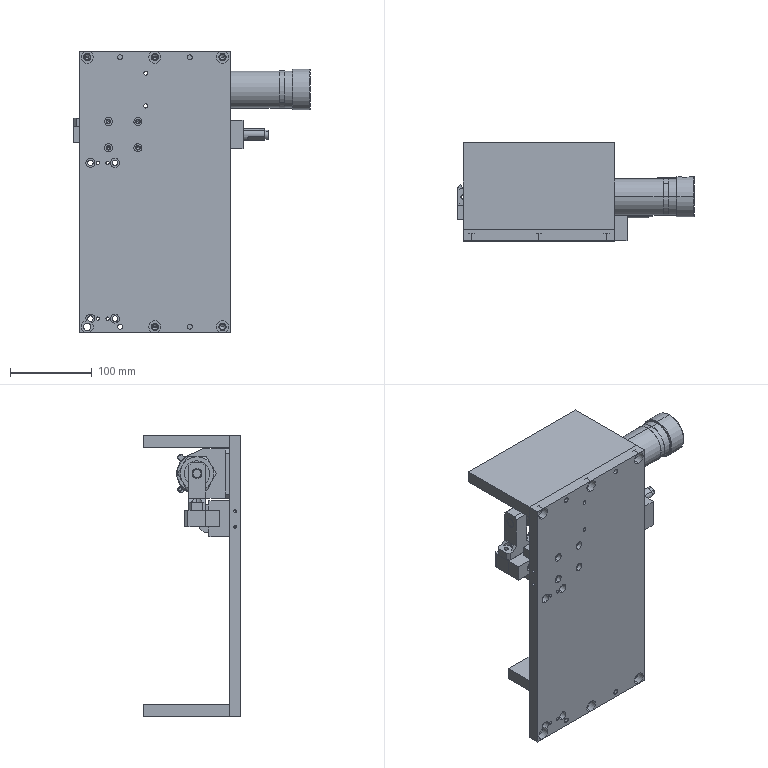Assembly | SolidWorks | mm | 19 component files | 19 solids | 807 faces | box 288.5 x 119.4 x 344 mm | volume 1839364 mm3 | plane 357 | cylinder 309 | cone 109 | torus 28 | sphere 4 | commonest cylinder face diameters 6.8 x26 6 x26 10 x18 5.5 x18 4.2 x18 11 x14 21.289 x14 45 x12
Bill of materials:
40_M12x1_25_Nut | 1 |  | Hexagonal prism with a central cylindrical through-bore and chamfered corners on both faces; looks like a hex nut.
ACA_1412_1_NT | 2 |  | Thin hexagonal prism with a large central through-bore and chamfered edges; looks like a thin hex nut or a hex ring.
ACA_1412_2_N_Body | 1 |  | Long stepped cylindrical body: a small-diameter pin at one end, narrow circumferential grooves next to it, a main cylindrical body with a long flat along part of its length, and a reduced-diameter end with a small central hole.
BufferFixingBlock | 1 |  | Rectangular block with one large through-hole and two smaller through-holes, plus two chamfered corners at one end.
CS1_M_A40 | 2 |  | Thin circular band loop joined to a rectangular housing block, with a stepped cylindrical shank sticking out of the housing; looks like a band-style clamp.
FlipMechanismA-08 | 1 |  | T-shaped support block: an upright with one transverse through-hole on a base flange with two mounting holes, chamfered corners, and an arched cutout under the upright.
FlipMechanismA-17 | 1 |  | Thin rectangular plate with many through-holes of mixed sizes, grouped near the two short ends and in an upper cluster, plus two small holes in one narrow edge.
FlipMechanismB-09 | 1 |  | L-shaped bent plate bracket: one leg has two small holes and chamfered corners; the other leg has one large hole and a rounded end.
FlipMechanismB-10 | 1 |  | Flat rectangular plate with plain top and bottom faces and several holes drilled into its edges.
FlipMechanismB-20 | 1 |  | Nearly square flat plate with two holes drilled into one edge.
FloatingJointSMCJA40-12-175 | 1 |  | Stepped cylindrical part: a large central cylinder, a small chamfered pin on one side with a short neck that has flats, and a smaller hollow tubular extension with a central bore on the other side.
GuideRailHIWINHGH20CA1R220-Z0-C | 1 |  | Long rectangular bar with three evenly spaced circular through-holes passing through one pair of faces.
MAL_40x75_S_U_c | 1 |  | Elongated cylindrical body of revolution with a slightly larger collar at each end and a short, smaller-diameter coaxial boss at one end.
MAL_40x75_S_U_r | 1 |  | Slender stepped shaft ending in a short, larger-diameter disc head with two circumferential grooves.
MAL40_M30x2_Nut | 1 |  | Thin hexagonal ring shaped like a jam nut, with a large central round through-bore and chamfered corners on one face.
RackAModule2.0 | 1 |  | Rectangular bar with a row of triangular teeth cut along part of one long edge, plus transverse holes in two perpendicular faces.
SliderHIWINHGH20CA | 1 |  | Rectangular block with a rectangular channel running its full length along one face, giving a C-shaped cross-section, and four holes on a large face.
Mates:
1. coincident | MAL_40x75_S_U_c-1 axis at (-80.9, 0, 0) dir (1, 0, 0) | MAL_40x75_S_U_r-1 axis at (65.65, 0, 0) dir (-1, 0, 0)
2. coincident | MAL_40x75_S_U_c-1 axis at (-80.9, 0, 0) dir (1, 0, 0) | MAL_40x75_S_U_r-1 axis at (65.65, 0, 0) dir (-1, 0, 0)
3. coincident | MAL_40x75_S_U_c-1 axis at (-80.9, 0, 0) dir (1, 0, 0) | MAL_40x75_S_U_r-1 axis at (65.65, 0, 0) dir (-1, 0, 0)
4. angle | MAL_40x75_S_U_r-1 plane at (-15.25, 0, 0) dir (0, 0, -1) | MAL_40x75_S_U_c-1 plane at (0, 0, 0) dir (0, 0, -1)
5. coincident | MAL_40x75_S_U_c-1 axis at (-80.9, 0, 0) dir (1, 0, 0) | MAL40_M30x2_Nut-1 axis at (66.9, 0, 0) dir (-1, 0, 0)
6. coincident | MAL_40x75_S_U_c-1 axis at (-80.9, 0, 0) dir (1, 0, 0) | MAL40_M30x2_Nut-1 axis at (66.9, 0, 0) dir (-1, 0, 0)
7. coincident | MAL_40x75_S_U_c-1 axis at (-80.9, 0, 0) dir (1, 0, 0) | MAL40_M30x2_Nut-1 axis at (66.9, 0, 0) dir (-1, 0, 0)
8. angle | MAL40_M30x2_Nut-1 plane at (-14, 0, 0) dir (0, 0, -1) | MAL_40x75_S_U_c-1 plane at (0, 0, 0) dir (0, 0, -1)
9. distance | 40_M12x1_25_Nut-1 plane at (-44.25, 0, 0) dir (1, 0, 0) | MAL_40x75_S_U_c-1 plane at (-34, 0, 0) dir (-1, 0, 0)
10. coincident | MAL_40x75_S_U_c-1 axis at (-80.9, 0, 0) dir (1, 0, 0) | 40_M12x1_25_Nut-1 axis at (33.15, 0, 0) dir (-1, 0, 0)
11. coincident | MAL_40x75_S_U_c-1 axis at (-80.9, 0, 0) dir (1, 0, 0) | 40_M12x1_25_Nut-1 axis at (33.15, 0, 0) dir (-1, 0, 0)
12. coincident | MAL_40x75_S_U_c-1 axis at (-80.9, 0, 0) dir (1, 0, 0) | 40_M12x1_25_Nut-1 axis at (33.15, 0, 0) dir (-1, 0, 0)
13. angle | 40_M12x1_25_Nut-1 plane at (-47.75, 0, 0) dir (0, 0, -1) | MAL_40x75_S_U_c-1 plane at (0, 0, 0) dir (0, 0, -1)
14. distance | CS1_M_A40-1 plane at (23, 0, 0) dir (1, 0, 0) | MAL_40x75_S_U_c-1 plane at (23, 0, 0) dir (-1, 0, 0)
15. coincident | MAL_40x75_S_U_c-1 axis at (-80.9, 0, 0) dir (1, 0, 0) | CS1_M_A40-1 axis at (103.9, 0, 0) dir (-1, 0, 0)
16. coincident | MAL_40x75_S_U_c-1 axis at (-80.9, 0, 0) dir (1, 0, 0) | CS1_M_A40-1 axis at (103.9, 0, 0) dir (-1, 0, 0)
17. coincident | MAL_40x75_S_U_c-1 axis at (-80.9, 0, 0) dir (1, 0, 0) | CS1_M_A40-1 axis at (103.9, 0, 0) dir (-1, 0, 0)
18. angle | CS1_M_A40-1 plane at (23, 0, 0) dir (0, 0.7071, -0.7071) | MAL_40x75_S_U_c-1 plane at (0, 0, 0) dir (0, 0, -1)
19. distance | CS1_M_A40-2 plane at (144, 0, 0) dir (-1, 0, 0) | MAL_40x75_S_U_c-1 plane at (144, 0, 0) dir (1, 0, 0)
20. coincident | MAL_40x75_S_U_c-1 axis at (80.9, 0, 0) dir (-1, 0, 0) | CS1_M_A40-2 axis at (63.1, 0, 0) dir (1, 0, 0)
21. coincident | MAL_40x75_S_U_c-1 axis at (80.9, 0, 0) dir (-1, 0, 0) | CS1_M_A40-2 axis at (63.1, 0, 0) dir (1, 0, 0)
22. coincident | MAL_40x75_S_U_c-1 axis at (80.9, 0, 0) dir (-1, 0, 0) | CS1_M_A40-2 axis at (63.1, 0, 0) dir (1, 0, 0)
23. angle | CS1_M_A40-2 plane at (144, 0, 0) dir (0, 0.7071, 0.7071) | MAL_40x75_S_U_c-1 plane at (0, 0, 0) dir (0, 0, -1)
24. coincident | RackAModule2.0-1 face at (-121.5, -10, -45) dir (0, 0, 1) | FlipMechanismA-08-1 face at (-121.5, -10, -45) dir (0, 0, -1)
25. coincident | GuideRailHIWINHGH20CA1R220-Z0-C-1 face at (38.5, -10, -45) dir (0, 1, 0) | FlipMechanismA-08-1 face at (-99, -10, -40) dir (0, -1, 0)
26. coincident | GuideRailHIWINHGH20CA1R220-Z0-C-1 face at (-121.5, -27.5, -65) dir (-1, 0, 0) | FlipMechanismA-08-1 face at (-121.5, -10, -45) dir (-1, 0, 0)
27. distance | SliderHIWINHGH20CA-1 face at (-100, -39.6, -77) dir (-1, 0, 0) | FlipMechanismA-17-1 face at (-115, -39.6, 47) dir (-1, 0, 0)
28. coincident | FlipMechanismA-17-1 face at (-22.5, -39.6, -125) dir (0, 1, 0) | FlipMechanismB-09-1 face at (-5, -39.6, 0) dir (0, -1, 0)
29. distance | FlipMechanismA-17-1 face at (70, -39.6, 47) dir (1, 0, 0) | FlipMechanismB-09-1 face at (0, -1.1, 0) dir (1, 0, 0)
30. distance | FlipMechanismB-09-1 face at (-5, -39.6, 30) dir (0, 0, 1) | FlipMechanismA-17-1 face at (70, -39.6, 47) dir (0, 0, 1)
31. coincident | SliderHIWINHGH20CA-1 face at (-100, -39.6, -77) dir (0, -1, 0) | FlipMechanismA-17-1 face at (-22.5, -39.6, -125) dir (0, 1, 0)
32. coincident | FlipMechanismA-17-1 face at (70, -39.6, 47) dir (0, 0, 1) | FlipMechanismB-10-1 face at (-22.5, 13.1, 47) dir (0, 0, 1)
33. coincident | FlipMechanismA-17-1 face at (-22.5, -39.6, -125) dir (0, 1, 0) | FlipMechanismB-10-1 face at (70, -39.6, 47) dir (0, -1, 0)
34. coincident | FlipMechanismA-17-1 face at (-115, -39.6, 47) dir (-1, 0, 0) | FlipMechanismB-10-1 face at (-115, -39.6, 47) dir (-1, 0, 0)
35. coincident | FlipMechanismA-17-1 face at (-22.5, -39.6, -125) dir (0, 1, 0) | FlipMechanismB-20-1 face at (70, -39.6, -297) dir (0, -1, 0)
36. coincident | FlipMechanismA-17-1 face at (70, -39.6, -297) dir (0, 0, -1) | FlipMechanismB-20-1 face at (12.5, 13.1, -297) dir (0, 0, -1)
37. coincident | FlipMechanismA-17-1 face at (70, -39.6, 47) dir (1, 0, 0) | FlipMechanismB-20-1 face at (70, 65.8, -297) dir (1, 0, 0)
38. distance | GuideRailHIWINHGH20CA1R220-Z0-C-1 face at (-121.5, -27.5, -65) dir (-1, 0, 0) | FlipMechanismA-17-1 face at (-115, -39.6, 47) dir (-1, 0, 0)
39. coincident | RackAModule2.0-1 face at (-27.255, -10, -65) dir (0, -1, 0) | GuideRailHIWINHGH20CA1R220-Z0-C-1 face at (38.5, -10, -45) dir (0, 1, 0)
40. coincident | RackAModule2.0-1 face at (-121.5, -10, -45) dir (0, 0, 1) | GuideRailHIWINHGH20CA1R220-Z0-C-1 face at (38.5, -27.5, -45) dir (0, 0, 1)
41. coincident | RackAModule2.0-1 face at (-121.5, -10, -65) dir (-1, 0, 0) | GuideRailHIWINHGH20CA1R220-Z0-C-1 face at (-121.5, -27.5, -65) dir (-1, 0, 0)
42. coincident | GuideRailHIWINHGH20CA1R220-Z0-C-1 face at (38.5, -27.5, -45) dir (0, -1, 0) | SliderHIWINHGH20CA-1 face at (-100, -27.5, -65) dir (0, 1, 0)
43. coincident | GuideRailHIWINHGH20CA1R220-Z0-C-1 face at (38.5, -27.5, -45) dir (0, -1, 0) | SliderHIWINHGH20CA-1 face at (-100, -27.5, -65) dir (0, 1, 0)
44. coincident | GuideRailHIWINHGH20CA1R220-Z0-C-1 plane at (-41.5, -10, -55) dir (0, 0, 1) | SliderHIWINHGH20CA-1 plane at (-61.25, -27.5, -55) dir (0, 0, 1)
45. coincident | FlipMechanismA-17-1 face at (70, -39.6, 47) dir (1, 0, 0) | BufferFixingBlock-1 face at (70, -28.6, -55) dir (-1, 0, 0)
46. distance | BufferFixingBlock-1 plane at (85, -28.6, -55) dir (0, 0, -1) | GuideRailHIWINHGH20CA1R220-Z0-C-1 face at (38.5, -27.5, -65) dir (0, 0, -1)
47. coincident | FlipMechanismA-17-1 face at (-22.5, -53.6, -125) dir (0, -1, 0) | BufferFixingBlock-1 face at (70, -53.6, -42.5) dir (0, -1, 0)
48. coincident | BufferFixingBlock-1 face at (70, -28.6, -55) dir (-1, 0, 0) | BufferAIRTACACA_1412_2_N-1/ACA_1412_1_NT-1 face at (70, -23.054, -60.4) dir (1, 0, 0)
49. concentric | MAL_40x75_S_U_r-1 face at (115.75, 0, 0) dir (-1, 0, 0) r 6 | FloatingJointSMCJA40-12-175-1 face at (-53.25, 0, 0) dir (1, 0, 0) r 10.333
50. distance | FloatingJointSMCJA40-12-175-1 face at (-47.75, -7.544, -3.128) dir (1, 0, 0) | 40_M12x1_25_Nut-1 face at (-47.75, 0, 0) dir (-1, 0, 0)
51. concentric | BufferFixingBlock-1 face at (85, -18.6, -55) dir (-1, 0, 0) r 7 | BufferAIRTACACA_1412_2_N-1/ACA_1412_2_N_Body-1 face at (116.5, -18.6, -55) dir (-1, 0, 0) r 7
52. distance | ACA_1412_1_NT-1 plane at (0, 52.5, 0) dir (0, -1, 0) | ACA_1412_2_N_Body-1 plane at (0, 52.5, 0) dir (0, 1, 0)
53. coincident | ACA_1412_2_N_Body-1 axis at (0, 50, 0) dir (0, -1, 0) | ACA_1412_1_NT-1 axis at (0, -3.5, 0) dir (0, 1, 0)
54. coincident | ACA_1412_2_N_Body-1 axis at (0, 50, 0) dir (0, -1, 0) | ACA_1412_1_NT-1 axis at (0, -3.5, 0) dir (0, 1, 0)
55. coincident | ACA_1412_2_N_Body-1 axis at (0, 50, 0) dir (0, -1, 0) | ACA_1412_1_NT-1 axis at (0, -3.5, 0) dir (0, 1, 0)
56. angle | ACA_1412_1_NT-1 plane at (0, 46.5, 0) dir (1, 0, 0) | ACA_1412_2_N_Body-1 plane at (0, 0, 0) dir (1, 0, 0)
57. distance | ACA_1412_1_NT-2 plane at (0, 58.5, 0) dir (0, -1, 0) | ACA_1412_2_N_Body-1 plane at (0, 52.5, 0) dir (0, 1, 0)
58. coincident | ACA_1412_2_N_Body-1 axis at (0, 50, 0) dir (0, -1, 0) | ACA_1412_1_NT-2 axis at (0, 2.5, 0) dir (0, 1, 0)
59. coincident | ACA_1412_2_N_Body-1 axis at (0, 50, 0) dir (0, -1, 0) | ACA_1412_1_NT-2 axis at (0, 2.5, 0) dir (0, 1, 0)
60. coincident | ACA_1412_2_N_Body-1 axis at (0, 50, 0) dir (0, -1, 0) | ACA_1412_1_NT-2 axis at (0, 2.5, 0) dir (0, 1, 0)
61. angle | ACA_1412_1_NT-2 plane at (0, 52.5, 0) dir (1, 0, 0) | ACA_1412_2_N_Body-1 plane at (0, 0, 0) dir (1, 0, 0)